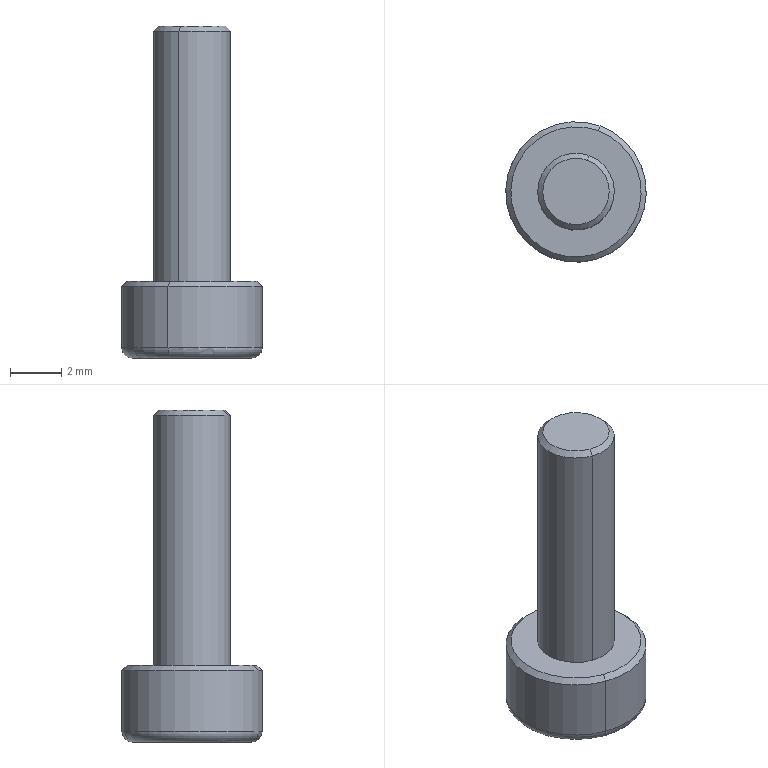Component | SolidWorks | SocketHeadCapScrew_M3_10-4 | 1 solid | 20 faces | box 5.5 x 5.5 x 13 mm | volume 134 mm3 | plane 10 | cone 4 | cylinder 4 | torus 2 | commonest cylinder face diameters 5.5 x2 3 x2
STEP:
#1=COLOUR_RGB('',0.7922,0.8196,0.9333);
#2=FILL_AREA_STYLE_COLOUR('',#1);
#3=FILL_AREA_STYLE('',(#2));
#4=SURFACE_STYLE_FILL_AREA(#3);
#5=SURFACE_SIDE_STYLE('',(#4));
#6=SURFACE_STYLE_USAGE(.BOTH.,#5);
#7=PRESENTATION_STYLE_ASSIGNMENT((#6));
#8=CARTESIAN_POINT('',(-0.4112,0.1684,-0.6711));
#9=VERTEX_POINT('',#8);
#10=CARTESIAN_POINT('',(-0.3762,0.2646,-0.6711));
#11=VERTEX_POINT('',#10);
#12=CARTESIAN_POINT('',(-0.3937,0.2165,-0.6711));
#13=DIRECTION('',(-0.,-0.,1.));
#14=DIRECTION('',(0.3419,0.9397,0.));
#15=AXIS2_PLACEMENT_3D('',#12,#13,#14);
#16=CIRCLE('',#15,0.05118);
#17=EDGE_CURVE('',#9,#11,#16,.T.);
#18=ORIENTED_EDGE('',*,*,#17,.F.);
#19=CARTESIAN_POINT('',(-0.4139,0.161,-0.679));
#20=VERTEX_POINT('',#19);
#21=CARTESIAN_POINT('',(-0.4139,0.161,-0.679));
#22=DIRECTION('',(-0.2417,-0.6645,-0.7071));
#23=VECTOR('',#22,39.37);
#24=LINE('',#21,#23);
#25=EDGE_CURVE('',#9,#20,#24,.T.);
#26=ORIENTED_EDGE('',*,*,#25,.T.);
#27=CARTESIAN_POINT('',(-0.3735,0.272,-0.679));
#28=VERTEX_POINT('',#27);
#29=CARTESIAN_POINT('',(-0.3937,0.2165,-0.679));
#30=DIRECTION('',(0.,0.,-1.));
#31=DIRECTION('',(0.3419,0.9397,0.));
#32=AXIS2_PLACEMENT_3D('',#29,#30,#31);
#33=CIRCLE('',#32,0.05906);
#34=EDGE_CURVE('',#28,#20,#33,.T.);
#35=ORIENTED_EDGE('',*,*,#34,.F.);
#36=CARTESIAN_POINT('',(-0.3735,0.272,-0.679));
#37=DIRECTION('',(0.2417,0.6645,-0.7071));
#38=VECTOR('',#37,39.37);
#39=LINE('',#36,#38);
#40=EDGE_CURVE('',#11,#28,#39,.T.);
#41=ORIENTED_EDGE('',*,*,#40,.F.);
#42=EDGE_LOOP('',(#18,#26,#35,#41));
#43=FACE_OUTER_BOUND('',#42,.T.);
#44=CARTESIAN_POINT('',(-0.3937,0.2165,-0.679));
#45=DIRECTION('',(0.,0.,-1.));
#46=DIRECTION('',(0.3419,0.9397,0.));
#47=AXIS2_PLACEMENT_3D('',#44,#45,#46);
#48=CONICAL_SURFACE('',#47,0.05906,0.7854);
#49=ADVANCED_FACE('',(#43),#48,.T.);
#50=CARTESIAN_POINT('',(-0.428,0.1222,-1.065));
#51=VERTEX_POINT('',#50);
#52=CARTESIAN_POINT('',(-0.3594,0.3109,-1.065));
#53=VERTEX_POINT('',#52);
#54=CARTESIAN_POINT('',(-0.3937,0.2165,-1.065));
#55=DIRECTION('',(-0.,-0.,1.));
#56=DIRECTION('',(0.3419,0.9397,0.));
#57=AXIS2_PLACEMENT_3D('',#54,#55,#56);
#58=CIRCLE('',#57,0.1004);
#59=EDGE_CURVE('',#51,#53,#58,.T.);
#60=ORIENTED_EDGE('',*,*,#59,.F.);
#61=CARTESIAN_POINT('',(-0.4307,0.1148,-1.073));
#62=VERTEX_POINT('',#61);
#63=CARTESIAN_POINT('',(-0.4307,0.1148,-1.073));
#64=DIRECTION('',(-0.2417,-0.6645,-0.7071));
#65=VECTOR('',#64,39.37);
#66=LINE('',#63,#65);
#67=EDGE_CURVE('',#51,#62,#66,.T.);
#68=ORIENTED_EDGE('',*,*,#67,.T.);
#69=CARTESIAN_POINT('',(-0.3567,0.3183,-1.073));
#70=VERTEX_POINT('',#69);
#71=CARTESIAN_POINT('',(-0.3937,0.2165,-1.073));
#72=DIRECTION('',(0.,0.,-1.));
#73=DIRECTION('',(0.3419,0.9397,0.));
#74=AXIS2_PLACEMENT_3D('',#71,#72,#73);
#75=CIRCLE('',#74,0.1083);
#76=EDGE_CURVE('',#70,#62,#75,.T.);
#77=ORIENTED_EDGE('',*,*,#76,.F.);
#78=CARTESIAN_POINT('',(-0.3567,0.3183,-1.073));
#79=DIRECTION('',(0.2417,0.6645,-0.7071));
#80=VECTOR('',#79,39.37);
#81=LINE('',#78,#80);
#82=EDGE_CURVE('',#53,#70,#81,.T.);
#83=ORIENTED_EDGE('',*,*,#82,.F.);
#84=EDGE_LOOP('',(#60,#68,#77,#83));
#85=FACE_OUTER_BOUND('',#84,.T.);
#86=CARTESIAN_POINT('',(-0.3937,0.2165,-1.073));
#87=DIRECTION('',(0.,0.,-1.));
#88=DIRECTION('',(0.3419,0.9397,0.));
#89=AXIS2_PLACEMENT_3D('',#86,#87,#88);
#90=CONICAL_SURFACE('',#89,0.1083,0.7854);
#91=ADVANCED_FACE('',(#85),#90,.T.);
#92=CARTESIAN_POINT('',(-0.3567,0.3183,-1.167));
#93=VERTEX_POINT('',#92);
#94=CARTESIAN_POINT('',(-0.4307,0.1148,-1.167));
#95=VERTEX_POINT('',#94);
#96=CARTESIAN_POINT('',(-0.3937,0.2165,-1.167));
#97=DIRECTION('',(0.,0.,-1.));
#98=DIRECTION('',(0.3419,0.9397,0.));
#99=AXIS2_PLACEMENT_3D('',#96,#97,#98);
#100=CIRCLE('',#99,0.1083);
#101=EDGE_CURVE('',#93,#95,#100,.T.);
#102=ORIENTED_EDGE('',*,*,#101,.T.);
#103=CARTESIAN_POINT('',(-0.4253,0.1296,-1.183));
#104=VERTEX_POINT('',#103);
#105=CARTESIAN_POINT('',(-0.4253,0.1296,-1.167));
#106=DIRECTION('',(0.9397,-0.3419,-0.));
#107=DIRECTION('',(0.3419,0.9397,0.));
#108=AXIS2_PLACEMENT_3D('',#105,#106,#107);
#109=CIRCLE('',#108,0.01575);
#110=EDGE_CURVE('',#95,#104,#109,.T.);
#111=ORIENTED_EDGE('',*,*,#110,.T.);
#112=CARTESIAN_POINT('',(-0.3621,0.3035,-1.183));
#113=VERTEX_POINT('',#112);
#114=CARTESIAN_POINT('',(-0.3937,0.2165,-1.183));
#115=DIRECTION('',(0.,0.,-1.));
#116=DIRECTION('',(0.3419,0.9397,0.));
#117=AXIS2_PLACEMENT_3D('',#114,#115,#116);
#118=CIRCLE('',#117,0.09252);
#119=EDGE_CURVE('',#113,#104,#118,.T.);
#120=ORIENTED_EDGE('',*,*,#119,.F.);
#121=CARTESIAN_POINT('',(-0.3621,0.3035,-1.167));
#122=DIRECTION('',(-0.9397,0.3419,0.));
#123=DIRECTION('',(-0.3419,-0.9397,0.));
#124=AXIS2_PLACEMENT_3D('',#121,#122,#123);
#125=CIRCLE('',#124,0.01575);
#126=EDGE_CURVE('',#93,#113,#125,.T.);
#127=ORIENTED_EDGE('',*,*,#126,.F.);
#128=EDGE_LOOP('',(#102,#111,#120,#127));
#129=FACE_OUTER_BOUND('',#128,.T.);
#130=CARTESIAN_POINT('',(-0.3937,0.2165,-1.167));
#131=DIRECTION('',(0.,0.,-1.));
#132=DIRECTION('',(0.3419,0.9397,0.));
#133=AXIS2_PLACEMENT_3D('',#130,#131,#132);
#134=TOROIDAL_SURFACE('',#133,0.09252,0.01575);
#135=ADVANCED_FACE('',(#129),#134,.T.);
#136=ORIENTED_EDGE('',*,*,#76,.T.);
#137=CARTESIAN_POINT('',(-0.4307,0.1148,-1.196));
#138=DIRECTION('',(0.,0.,-1.));
#139=VECTOR('',#138,39.37);
#140=LINE('',#137,#139);
#141=EDGE_CURVE('',#62,#95,#140,.T.);
#142=ORIENTED_EDGE('',*,*,#141,.T.);
#143=ORIENTED_EDGE('',*,*,#101,.F.);
#144=CARTESIAN_POINT('',(-0.3567,0.3183,-1.196));
#145=DIRECTION('',(0.,0.,-1.));
#146=VECTOR('',#145,39.37);
#147=LINE('',#144,#146);
#148=EDGE_CURVE('',#70,#93,#147,.T.);
#149=ORIENTED_EDGE('',*,*,#148,.F.);
#150=EDGE_LOOP('',(#136,#142,#143,#149));
#151=FACE_OUTER_BOUND('',#150,.T.);
#152=CARTESIAN_POINT('',(-0.3937,0.2165,-1.196));
#153=DIRECTION('',(0.,0.,-1.));
#154=DIRECTION('',(0.3419,0.9397,0.));
#155=AXIS2_PLACEMENT_3D('',#152,#153,#154);
#156=CYLINDRICAL_SURFACE('',#155,0.1083);
#157=ADVANCED_FACE('',(#151),#156,.T.);
#158=ORIENTED_EDGE('',*,*,#34,.T.);
#159=CARTESIAN_POINT('',(-0.4139,0.161,-1.065));
#160=VERTEX_POINT('',#159);
#161=CARTESIAN_POINT('',(-0.4139,0.161,-1.196));
#162=DIRECTION('',(0.,0.,-1.));
#163=VECTOR('',#162,39.37);
#164=LINE('',#161,#163);
#165=EDGE_CURVE('',#20,#160,#164,.T.);
#166=ORIENTED_EDGE('',*,*,#165,.T.);
#167=CARTESIAN_POINT('',(-0.3735,0.272,-1.065));
#168=VERTEX_POINT('',#167);
#169=CARTESIAN_POINT('',(-0.3937,0.2165,-1.065));
#170=DIRECTION('',(0.,0.,-1.));
#171=DIRECTION('',(0.3419,0.9397,0.));
#172=AXIS2_PLACEMENT_3D('',#169,#170,#171);
#173=CIRCLE('',#172,0.05906);
#174=EDGE_CURVE('',#168,#160,#173,.T.);
#175=ORIENTED_EDGE('',*,*,#174,.F.);
#176=CARTESIAN_POINT('',(-0.3735,0.272,-1.196));
#177=DIRECTION('',(0.,0.,-1.));
#178=VECTOR('',#177,39.37);
#179=LINE('',#176,#178);
#180=EDGE_CURVE('',#28,#168,#179,.T.);
#181=ORIENTED_EDGE('',*,*,#180,.F.);
#182=EDGE_LOOP('',(#158,#166,#175,#181));
#183=FACE_OUTER_BOUND('',#182,.T.);
#184=CARTESIAN_POINT('',(-0.3937,0.2165,-1.196));
#185=DIRECTION('',(0.,0.,-1.));
#186=DIRECTION('',(0.3419,0.9397,0.));
#187=AXIS2_PLACEMENT_3D('',#184,#185,#186);
#188=CYLINDRICAL_SURFACE('',#187,0.05906);
#189=ADVANCED_FACE('',(#183),#188,.T.);
#190=CARTESIAN_POINT('',(-0.3937,0.2165,-0.6711));
#191=DIRECTION('',(-0.,-0.,1.));
#192=DIRECTION('',(0.3419,0.9397,0.));
#193=AXIS2_PLACEMENT_3D('',#190,#191,#192);
#194=CIRCLE('',#193,0.05118);
#195=EDGE_CURVE('',#11,#9,#194,.T.);
#196=ORIENTED_EDGE('',*,*,#195,.T.);
#197=ORIENTED_EDGE('',*,*,#17,.T.);
#198=EDGE_LOOP('',(#196,#197));
#199=FACE_OUTER_BOUND('',#198,.T.);
#200=CARTESIAN_POINT('',(-0.3382,0.1963,-0.6711));
#201=DIRECTION('',(0.,0.,-1.));
#202=DIRECTION('',(0.3419,0.9397,0.));
#203=AXIS2_PLACEMENT_3D('',#200,#201,#202);
#204=PLANE('',#203);
#205=ADVANCED_FACE('',(#199),#204,.F.);
#206=ORIENTED_EDGE('',*,*,#165,.F.);
#207=CARTESIAN_POINT('',(-0.3937,0.2165,-0.679));
#208=DIRECTION('',(0.,0.,-1.));
#209=DIRECTION('',(0.3419,0.9397,0.));
#210=AXIS2_PLACEMENT_3D('',#207,#208,#209);
#211=CIRCLE('',#210,0.05906);
#212=EDGE_CURVE('',#20,#28,#211,.T.);
#213=ORIENTED_EDGE('',*,*,#212,.T.);
#214=ORIENTED_EDGE('',*,*,#180,.T.);
#215=CARTESIAN_POINT('',(-0.3937,0.2165,-1.065));
#216=DIRECTION('',(0.,0.,-1.));
#217=DIRECTION('',(0.3419,0.9397,0.));
#218=AXIS2_PLACEMENT_3D('',#215,#216,#217);
#219=CIRCLE('',#218,0.05906);
#220=EDGE_CURVE('',#160,#168,#219,.T.);
#221=ORIENTED_EDGE('',*,*,#220,.F.);
#222=EDGE_LOOP('',(#206,#213,#214,#221));
#223=FACE_OUTER_BOUND('',#222,.T.);
#224=CARTESIAN_POINT('',(-0.3937,0.2165,-1.196));
#225=DIRECTION('',(0.,0.,-1.));
#226=DIRECTION('',(0.3419,0.9397,0.));
#227=AXIS2_PLACEMENT_3D('',#224,#225,#226);
#228=CYLINDRICAL_SURFACE('',#227,0.05906);
#229=ADVANCED_FACE('',(#223),#228,.T.);
#230=CARTESIAN_POINT('',(-0.3937,0.2165,-1.065));
#231=DIRECTION('',(-0.,-0.,1.));
#232=DIRECTION('',(0.3419,0.9397,0.));
#233=AXIS2_PLACEMENT_3D('',#230,#231,#232);
#234=CIRCLE('',#233,0.1004);
#235=EDGE_CURVE('',#53,#51,#234,.T.);
#236=ORIENTED_EDGE('',*,*,#235,.T.);
#237=ORIENTED_EDGE('',*,*,#59,.T.);
#238=EDGE_LOOP('',(#236,#237));
#239=FACE_OUTER_BOUND('',#238,.T.);
#240=ORIENTED_EDGE('',*,*,#174,.T.);
#241=ORIENTED_EDGE('',*,*,#220,.T.);
#242=EDGE_LOOP('',(#240,#241));
#243=FACE_BOUND('',#242,.T.);
#244=CARTESIAN_POINT('',(-0.292,0.1795,-1.065));
#245=DIRECTION('',(0.,0.,-1.));
#246=DIRECTION('',(0.3419,0.9397,0.));
#247=AXIS2_PLACEMENT_3D('',#244,#245,#246);
#248=PLANE('',#247);
#249=ADVANCED_FACE('',(#239,#243),#248,.F.);
#250=ORIENTED_EDGE('',*,*,#141,.F.);
#251=CARTESIAN_POINT('',(-0.3937,0.2165,-1.073));
#252=DIRECTION('',(0.,0.,-1.));
#253=DIRECTION('',(0.3419,0.9397,0.));
#254=AXIS2_PLACEMENT_3D('',#251,#252,#253);
#255=CIRCLE('',#254,0.1083);
#256=EDGE_CURVE('',#62,#70,#255,.T.);
#257=ORIENTED_EDGE('',*,*,#256,.T.);
#258=ORIENTED_EDGE('',*,*,#148,.T.);
#259=CARTESIAN_POINT('',(-0.3937,0.2165,-1.167));
#260=DIRECTION('',(0.,0.,-1.));
#261=DIRECTION('',(0.3419,0.9397,0.));
#262=AXIS2_PLACEMENT_3D('',#259,#260,#261);
#263=CIRCLE('',#262,0.1083);
#264=EDGE_CURVE('',#95,#93,#263,.T.);
#265=ORIENTED_EDGE('',*,*,#264,.F.);
#266=EDGE_LOOP('',(#250,#257,#258,#265));
#267=FACE_OUTER_BOUND('',#266,.T.);
#268=CARTESIAN_POINT('',(-0.3937,0.2165,-1.196));
#269=DIRECTION('',(0.,0.,-1.));
#270=DIRECTION('',(0.3419,0.9397,0.));
#271=AXIS2_PLACEMENT_3D('',#268,#269,#270);
#272=CYLINDRICAL_SURFACE('',#271,0.1083);
#273=ADVANCED_FACE('',(#267),#272,.T.);
#274=ORIENTED_EDGE('',*,*,#110,.F.);
#275=ORIENTED_EDGE('',*,*,#264,.T.);
#276=ORIENTED_EDGE('',*,*,#126,.T.);
#277=CARTESIAN_POINT('',(-0.3937,0.2165,-1.183));
#278=DIRECTION('',(0.,0.,-1.));
#279=DIRECTION('',(0.3419,0.9397,0.));
#280=AXIS2_PLACEMENT_3D('',#277,#278,#279);
#281=CIRCLE('',#280,0.09252);
#282=EDGE_CURVE('',#104,#113,#281,.T.);
#283=ORIENTED_EDGE('',*,*,#282,.F.);
#284=EDGE_LOOP('',(#274,#275,#276,#283));
#285=FACE_OUTER_BOUND('',#284,.T.);
#286=CARTESIAN_POINT('',(-0.3937,0.2165,-1.167));
#287=DIRECTION('',(0.,0.,-1.));
#288=DIRECTION('',(0.3419,0.9397,0.));
#289=AXIS2_PLACEMENT_3D('',#286,#287,#288);
#290=TOROIDAL_SURFACE('',#289,0.09252,0.01575);
#291=ADVANCED_FACE('',(#285),#290,.T.);
#292=CARTESIAN_POINT('',(-0.3743,0.2699,-1.183));
#293=VERTEX_POINT('',#292);
#294=CARTESIAN_POINT('',(-0.3377,0.2264,-1.183));
#295=VERTEX_POINT('',#294);
#296=CARTESIAN_POINT('',(-0.3743,0.2699,-1.183));
#297=DIRECTION('',(0.6429,-0.7659,-0.));
#298=VECTOR('',#297,39.37);
#299=LINE('',#296,#298);
#300=EDGE_CURVE('',#293,#295,#299,.T.);
#301=ORIENTED_EDGE('',*,*,#300,.F.);
#302=CARTESIAN_POINT('',(-0.4302,0.2601,-1.183));
#303=VERTEX_POINT('',#302);
#304=CARTESIAN_POINT('',(-0.4302,0.2601,-1.183));
#305=DIRECTION('',(0.9848,0.1738,0.));
#306=VECTOR('',#305,39.37);
#307=LINE('',#304,#306);
#308=EDGE_CURVE('',#303,#293,#307,.T.);
#309=ORIENTED_EDGE('',*,*,#308,.F.);
#310=CARTESIAN_POINT('',(-0.4497,0.2067,-1.183));
#311=VERTEX_POINT('',#310);
#312=CARTESIAN_POINT('',(-0.4497,0.2067,-1.183));
#313=DIRECTION('',(0.3419,0.9397,0.));
#314=VECTOR('',#313,39.37);
#315=LINE('',#312,#314);
#316=EDGE_CURVE('',#311,#303,#315,.T.);
#317=ORIENTED_EDGE('',*,*,#316,.F.);
#318=CARTESIAN_POINT('',(-0.4131,0.1631,-1.183));
#319=VERTEX_POINT('',#318);
#320=CARTESIAN_POINT('',(-0.4131,0.1631,-1.183));
#321=DIRECTION('',(-0.6429,0.7659,0.));
#322=VECTOR('',#321,39.37);
#323=LINE('',#320,#322);
#324=EDGE_CURVE('',#319,#311,#323,.T.);
#325=ORIENTED_EDGE('',*,*,#324,.F.);
#326=CARTESIAN_POINT('',(-0.3572,0.173,-1.183));
#327=VERTEX_POINT('',#326);
#328=CARTESIAN_POINT('',(-0.3572,0.173,-1.183));
#329=DIRECTION('',(-0.9848,-0.1738,-0.));
#330=VECTOR('',#329,39.37);
#331=LINE('',#328,#330);
#332=EDGE_CURVE('',#327,#319,#331,.T.);
#333=ORIENTED_EDGE('',*,*,#332,.F.);
#334=CARTESIAN_POINT('',(-0.3377,0.2264,-1.183));
#335=DIRECTION('',(-0.3419,-0.9397,-0.));
#336=VECTOR('',#335,39.37);
#337=LINE('',#334,#336);
#338=EDGE_CURVE('',#295,#327,#337,.T.);
#339=ORIENTED_EDGE('',*,*,#338,.F.);
#340=EDGE_LOOP('',(#301,#309,#317,#325,#333,#339));
#341=FACE_BOUND('',#340,.T.);
#342=ORIENTED_EDGE('',*,*,#119,.T.);
#343=ORIENTED_EDGE('',*,*,#282,.T.);
#344=EDGE_LOOP('',(#342,#343));
#345=FACE_OUTER_BOUND('',#344,.T.);
#346=CARTESIAN_POINT('',(-0.3937,0.2165,-1.183));
#347=DIRECTION('',(-0.,-0.,1.));
#348=DIRECTION('',(-0.3419,-0.9397,-0.));
#349=AXIS2_PLACEMENT_3D('',#346,#347,#348);
#350=PLANE('',#349);
#351=ADVANCED_FACE('',(#341,#345),#350,.F.);
#352=ORIENTED_EDGE('',*,*,#308,.T.);
#353=CARTESIAN_POINT('',(-0.3743,0.2699,-1.132));
#354=VERTEX_POINT('',#353);
#355=CARTESIAN_POINT('',(-0.3743,0.2699,-1.132));
#356=DIRECTION('',(0.,0.,-1.));
#357=VECTOR('',#356,39.37);
#358=LINE('',#355,#357);
#359=EDGE_CURVE('',#354,#293,#358,.T.);
#360=ORIENTED_EDGE('',*,*,#359,.F.);
#361=CARTESIAN_POINT('',(-0.4302,0.2601,-1.132));
#362=VERTEX_POINT('',#361);
#363=CARTESIAN_POINT('',(-0.4302,0.2601,-1.132));
#364=DIRECTION('',(0.9848,0.1738,0.));
#365=VECTOR('',#364,39.37);
#366=LINE('',#363,#365);
#367=EDGE_CURVE('',#362,#354,#366,.T.);
#368=ORIENTED_EDGE('',*,*,#367,.F.);
#369=CARTESIAN_POINT('',(-0.4302,0.2601,-1.132));
#370=DIRECTION('',(0.,0.,-1.));
#371=VECTOR('',#370,39.37);
#372=LINE('',#369,#371);
#373=EDGE_CURVE('',#362,#303,#372,.T.);
#374=ORIENTED_EDGE('',*,*,#373,.T.);
#375=EDGE_LOOP('',(#352,#360,#368,#374));
#376=FACE_OUTER_BOUND('',#375,.T.);
#377=CARTESIAN_POINT('',(-0.4302,0.2601,-1.132));
#378=DIRECTION('',(-0.1738,0.9848,0.));
#379=DIRECTION('',(-0.9848,-0.1738,-0.));
#380=AXIS2_PLACEMENT_3D('',#377,#378,#379);
#381=PLANE('',#380);
#382=ADVANCED_FACE('',(#376),#381,.F.);
#383=ORIENTED_EDGE('',*,*,#316,.T.);
#384=ORIENTED_EDGE('',*,*,#373,.F.);
#385=CARTESIAN_POINT('',(-0.4497,0.2067,-1.132));
#386=VERTEX_POINT('',#385);
#387=CARTESIAN_POINT('',(-0.4497,0.2067,-1.132));
#388=DIRECTION('',(0.3419,0.9397,0.));
#389=VECTOR('',#388,39.37);
#390=LINE('',#387,#389);
#391=EDGE_CURVE('',#386,#362,#390,.T.);
#392=ORIENTED_EDGE('',*,*,#391,.F.);
#393=CARTESIAN_POINT('',(-0.4497,0.2067,-1.132));
#394=DIRECTION('',(0.,0.,-1.));
#395=VECTOR('',#394,39.37);
#396=LINE('',#393,#395);
#397=EDGE_CURVE('',#386,#311,#396,.T.);
#398=ORIENTED_EDGE('',*,*,#397,.T.);
#399=EDGE_LOOP('',(#383,#384,#392,#398));
#400=FACE_OUTER_BOUND('',#399,.T.);
#401=CARTESIAN_POINT('',(-0.4497,0.2067,-1.132));
#402=DIRECTION('',(-0.9397,0.3419,0.));
#403=DIRECTION('',(-0.3419,-0.9397,-0.));
#404=AXIS2_PLACEMENT_3D('',#401,#402,#403);
#405=PLANE('',#404);
#406=ADVANCED_FACE('',(#400),#405,.F.);
#407=ORIENTED_EDGE('',*,*,#324,.T.);
#408=ORIENTED_EDGE('',*,*,#397,.F.);
#409=CARTESIAN_POINT('',(-0.4131,0.1631,-1.132));
#410=VERTEX_POINT('',#409);
#411=CARTESIAN_POINT('',(-0.4131,0.1631,-1.132));
#412=DIRECTION('',(-0.6429,0.7659,0.));
#413=VECTOR('',#412,39.37);
#414=LINE('',#411,#413);
#415=EDGE_CURVE('',#410,#386,#414,.T.);
#416=ORIENTED_EDGE('',*,*,#415,.F.);
#417=CARTESIAN_POINT('',(-0.4131,0.1631,-1.132));
#418=DIRECTION('',(0.,0.,-1.));
#419=VECTOR('',#418,39.37);
#420=LINE('',#417,#419);
#421=EDGE_CURVE('',#410,#319,#420,.T.);
#422=ORIENTED_EDGE('',*,*,#421,.T.);
#423=EDGE_LOOP('',(#407,#408,#416,#422));
#424=FACE_OUTER_BOUND('',#423,.T.);
#425=CARTESIAN_POINT('',(-0.4131,0.1631,-1.132));
#426=DIRECTION('',(-0.7659,-0.6429,-0.));
#427=DIRECTION('',(0.6429,-0.7659,-0.));
#428=AXIS2_PLACEMENT_3D('',#425,#426,#427);
#429=PLANE('',#428);
#430=ADVANCED_FACE('',(#424),#429,.F.);
#431=ORIENTED_EDGE('',*,*,#332,.T.);
#432=ORIENTED_EDGE('',*,*,#421,.F.);
#433=CARTESIAN_POINT('',(-0.3572,0.173,-1.132));
#434=VERTEX_POINT('',#433);
#435=CARTESIAN_POINT('',(-0.3572,0.173,-1.132));
#436=DIRECTION('',(-0.9848,-0.1738,-0.));
#437=VECTOR('',#436,39.37);
#438=LINE('',#435,#437);
#439=EDGE_CURVE('',#434,#410,#438,.T.);
#440=ORIENTED_EDGE('',*,*,#439,.F.);
#441=CARTESIAN_POINT('',(-0.3572,0.173,-1.132));
#442=DIRECTION('',(0.,0.,-1.));
#443=VECTOR('',#442,39.37);
#444=LINE('',#441,#443);
#445=EDGE_CURVE('',#434,#327,#444,.T.);
#446=ORIENTED_EDGE('',*,*,#445,.T.);
#447=EDGE_LOOP('',(#431,#432,#440,#446));
#448=FACE_OUTER_BOUND('',#447,.T.);
#449=CARTESIAN_POINT('',(-0.3572,0.173,-1.132));
#450=DIRECTION('',(0.1738,-0.9848,-0.));
#451=DIRECTION('',(0.9848,0.1738,0.));
#452=AXIS2_PLACEMENT_3D('',#449,#450,#451);
#453=PLANE('',#452);
#454=ADVANCED_FACE('',(#448),#453,.F.);
#455=ORIENTED_EDGE('',*,*,#338,.T.);
#456=ORIENTED_EDGE('',*,*,#445,.F.);
#457=CARTESIAN_POINT('',(-0.3377,0.2264,-1.132));
#458=VERTEX_POINT('',#457);
#459=CARTESIAN_POINT('',(-0.3377,0.2264,-1.132));
#460=DIRECTION('',(-0.3419,-0.9397,-0.));
#461=VECTOR('',#460,39.37);
#462=LINE('',#459,#461);
#463=EDGE_CURVE('',#458,#434,#462,.T.);
#464=ORIENTED_EDGE('',*,*,#463,.F.);
#465=CARTESIAN_POINT('',(-0.3377,0.2264,-1.132));
#466=DIRECTION('',(0.,0.,-1.));
#467=VECTOR('',#466,39.37);
#468=LINE('',#465,#467);
#469=EDGE_CURVE('',#458,#295,#468,.T.);
#470=ORIENTED_EDGE('',*,*,#469,.T.);
#471=EDGE_LOOP('',(#455,#456,#464,#470));
#472=FACE_OUTER_BOUND('',#471,.T.);
#473=CARTESIAN_POINT('',(-0.3377,0.2264,-1.132));
#474=DIRECTION('',(0.9397,-0.3419,-0.));
#475=DIRECTION('',(0.3419,0.9397,0.));
#476=AXIS2_PLACEMENT_3D('',#473,#474,#475);
#477=PLANE('',#476);
#478=ADVANCED_FACE('',(#472),#477,.F.);
#479=ORIENTED_EDGE('',*,*,#300,.T.);
#480=ORIENTED_EDGE('',*,*,#469,.F.);
#481=CARTESIAN_POINT('',(-0.3743,0.2699,-1.132));
#482=DIRECTION('',(0.6429,-0.7659,-0.));
#483=VECTOR('',#482,39.37);
#484=LINE('',#481,#483);
#485=EDGE_CURVE('',#354,#458,#484,.T.);
#486=ORIENTED_EDGE('',*,*,#485,.F.);
#487=ORIENTED_EDGE('',*,*,#359,.T.);
#488=EDGE_LOOP('',(#479,#480,#486,#487));
#489=FACE_OUTER_BOUND('',#488,.T.);
#490=CARTESIAN_POINT('',(-0.3743,0.2699,-1.132));
#491=DIRECTION('',(0.7659,0.6429,0.));
#492=DIRECTION('',(-0.6429,0.7659,0.));
#493=AXIS2_PLACEMENT_3D('',#490,#491,#492);
#494=PLANE('',#493);
#495=ADVANCED_FACE('',(#489),#494,.F.);
#496=ORIENTED_EDGE('',*,*,#367,.T.);
#497=ORIENTED_EDGE('',*,*,#485,.T.);
#498=ORIENTED_EDGE('',*,*,#463,.T.);
#499=ORIENTED_EDGE('',*,*,#439,.T.);
#500=ORIENTED_EDGE('',*,*,#415,.T.);
#501=ORIENTED_EDGE('',*,*,#391,.T.);
#502=EDGE_LOOP('',(#496,#497,#498,#499,#500,#501));
#503=FACE_OUTER_BOUND('',#502,.T.);
#504=CARTESIAN_POINT('',(-0.3183,0.2798,-1.132));
#505=DIRECTION('',(0.,0.,-1.));
#506=DIRECTION('',(0.3419,0.9397,0.));
#507=AXIS2_PLACEMENT_3D('',#504,#505,#506);
#508=PLANE('',#507);
#509=ADVANCED_FACE('',(#503),#508,.T.);
#510=ORIENTED_EDGE('',*,*,#67,.F.);
#511=ORIENTED_EDGE('',*,*,#235,.F.);
#512=ORIENTED_EDGE('',*,*,#82,.T.);
#513=ORIENTED_EDGE('',*,*,#256,.F.);
#514=EDGE_LOOP('',(#510,#511,#512,#513));
#515=FACE_OUTER_BOUND('',#514,.T.);
#516=CARTESIAN_POINT('',(-0.3937,0.2165,-1.073));
#517=DIRECTION('',(0.,0.,-1.));
#518=DIRECTION('',(0.3419,0.9397,0.));
#519=AXIS2_PLACEMENT_3D('',#516,#517,#518);
#520=CONICAL_SURFACE('',#519,0.1083,0.7854);
#521=ADVANCED_FACE('',(#515),#520,.T.);
#522=ORIENTED_EDGE('',*,*,#25,.F.);
#523=ORIENTED_EDGE('',*,*,#195,.F.);
#524=ORIENTED_EDGE('',*,*,#40,.T.);
#525=ORIENTED_EDGE('',*,*,#212,.F.);
#526=EDGE_LOOP('',(#522,#523,#524,#525));
#527=FACE_OUTER_BOUND('',#526,.T.);
#528=CARTESIAN_POINT('',(-0.3937,0.2165,-0.679));
#529=DIRECTION('',(0.,0.,-1.));
#530=DIRECTION('',(0.3419,0.9397,0.));
#531=AXIS2_PLACEMENT_3D('',#528,#529,#530);
#532=CONICAL_SURFACE('',#531,0.05906,0.7854);
#533=ADVANCED_FACE('',(#527),#532,.T.);
#534=CLOSED_SHELL('',(#49,#91,#135,#157,#189,#205,#229,#249,#273,#291,#351,#382,#406,#430,#454,#478,#495,#509,#521,#533));
#535=MANIFOLD_SOLID_BREP('',#534);
#536=STYLED_ITEM('',(#7),#535);
#537=(LENGTH_UNIT()NAMED_UNIT(*)SI_UNIT($,.METRE.));
#538=LENGTH_MEASURE_WITH_UNIT(LENGTH_MEASURE(0.0254),#537);
#539=DIMENSIONAL_EXPONENTS(1.,0.,0.,0.,0.,0.,0.);
#540=(CONVERSION_BASED_UNIT('',#538)LENGTH_UNIT()NAMED_UNIT(#539));
#541=UNCERTAINTY_MEASURE_WITH_UNIT(LENGTH_MEASURE(0.00001),#540,'','');
#542=(NAMED_UNIT(*)PLANE_ANGLE_UNIT()SI_UNIT($,.RADIAN.));
#543=(NAMED_UNIT(*)SI_UNIT($,.STERADIAN.)SOLID_ANGLE_UNIT());
#544=(GEOMETRIC_REPRESENTATION_CONTEXT(3)GLOBAL_UNCERTAINTY_ASSIGNED_CONTEXT((#541))GLOBAL_UNIT_ASSIGNED_CONTEXT((#540,#542,#543))REPRESENTATION_CONTEXT('',''));
#545=MECHANICAL_DESIGN_GEOMETRIC_PRESENTATION_REPRESENTATION('',(#536),#544);
#546=PRESENTATION_LAYER_ASSIGNMENT('','',(#536));
#547=CARTESIAN_POINT('',(0.,0.,0.));
#548=DIRECTION('',(0.,0.,1.));
#549=DIRECTION('',(1.,0.,0.));
#550=AXIS2_PLACEMENT_3D('',#547,#548,#549);
#551=(LENGTH_UNIT()NAMED_UNIT(*)SI_UNIT($,.METRE.));
#552=LENGTH_MEASURE_WITH_UNIT(LENGTH_MEASURE(0.0254),#551);
#553=DIMENSIONAL_EXPONENTS(1.,0.,0.,0.,0.,0.,0.);
#554=(CONVERSION_BASED_UNIT('',#552)LENGTH_UNIT()NAMED_UNIT(#553));
#555=UNCERTAINTY_MEASURE_WITH_UNIT(LENGTH_MEASURE(0.00001),#554,'','');
#556=(NAMED_UNIT(*)PLANE_ANGLE_UNIT()SI_UNIT($,.RADIAN.));
#557=(NAMED_UNIT(*)SI_UNIT($,.STERADIAN.)SOLID_ANGLE_UNIT());
#558=(GEOMETRIC_REPRESENTATION_CONTEXT(3)GLOBAL_UNCERTAINTY_ASSIGNED_CONTEXT((#555))GLOBAL_UNIT_ASSIGNED_CONTEXT((#554,#556,#557))REPRESENTATION_CONTEXT('',''));
#559=ADVANCED_BREP_SHAPE_REPRESENTATION('',(#535,#550),#558);